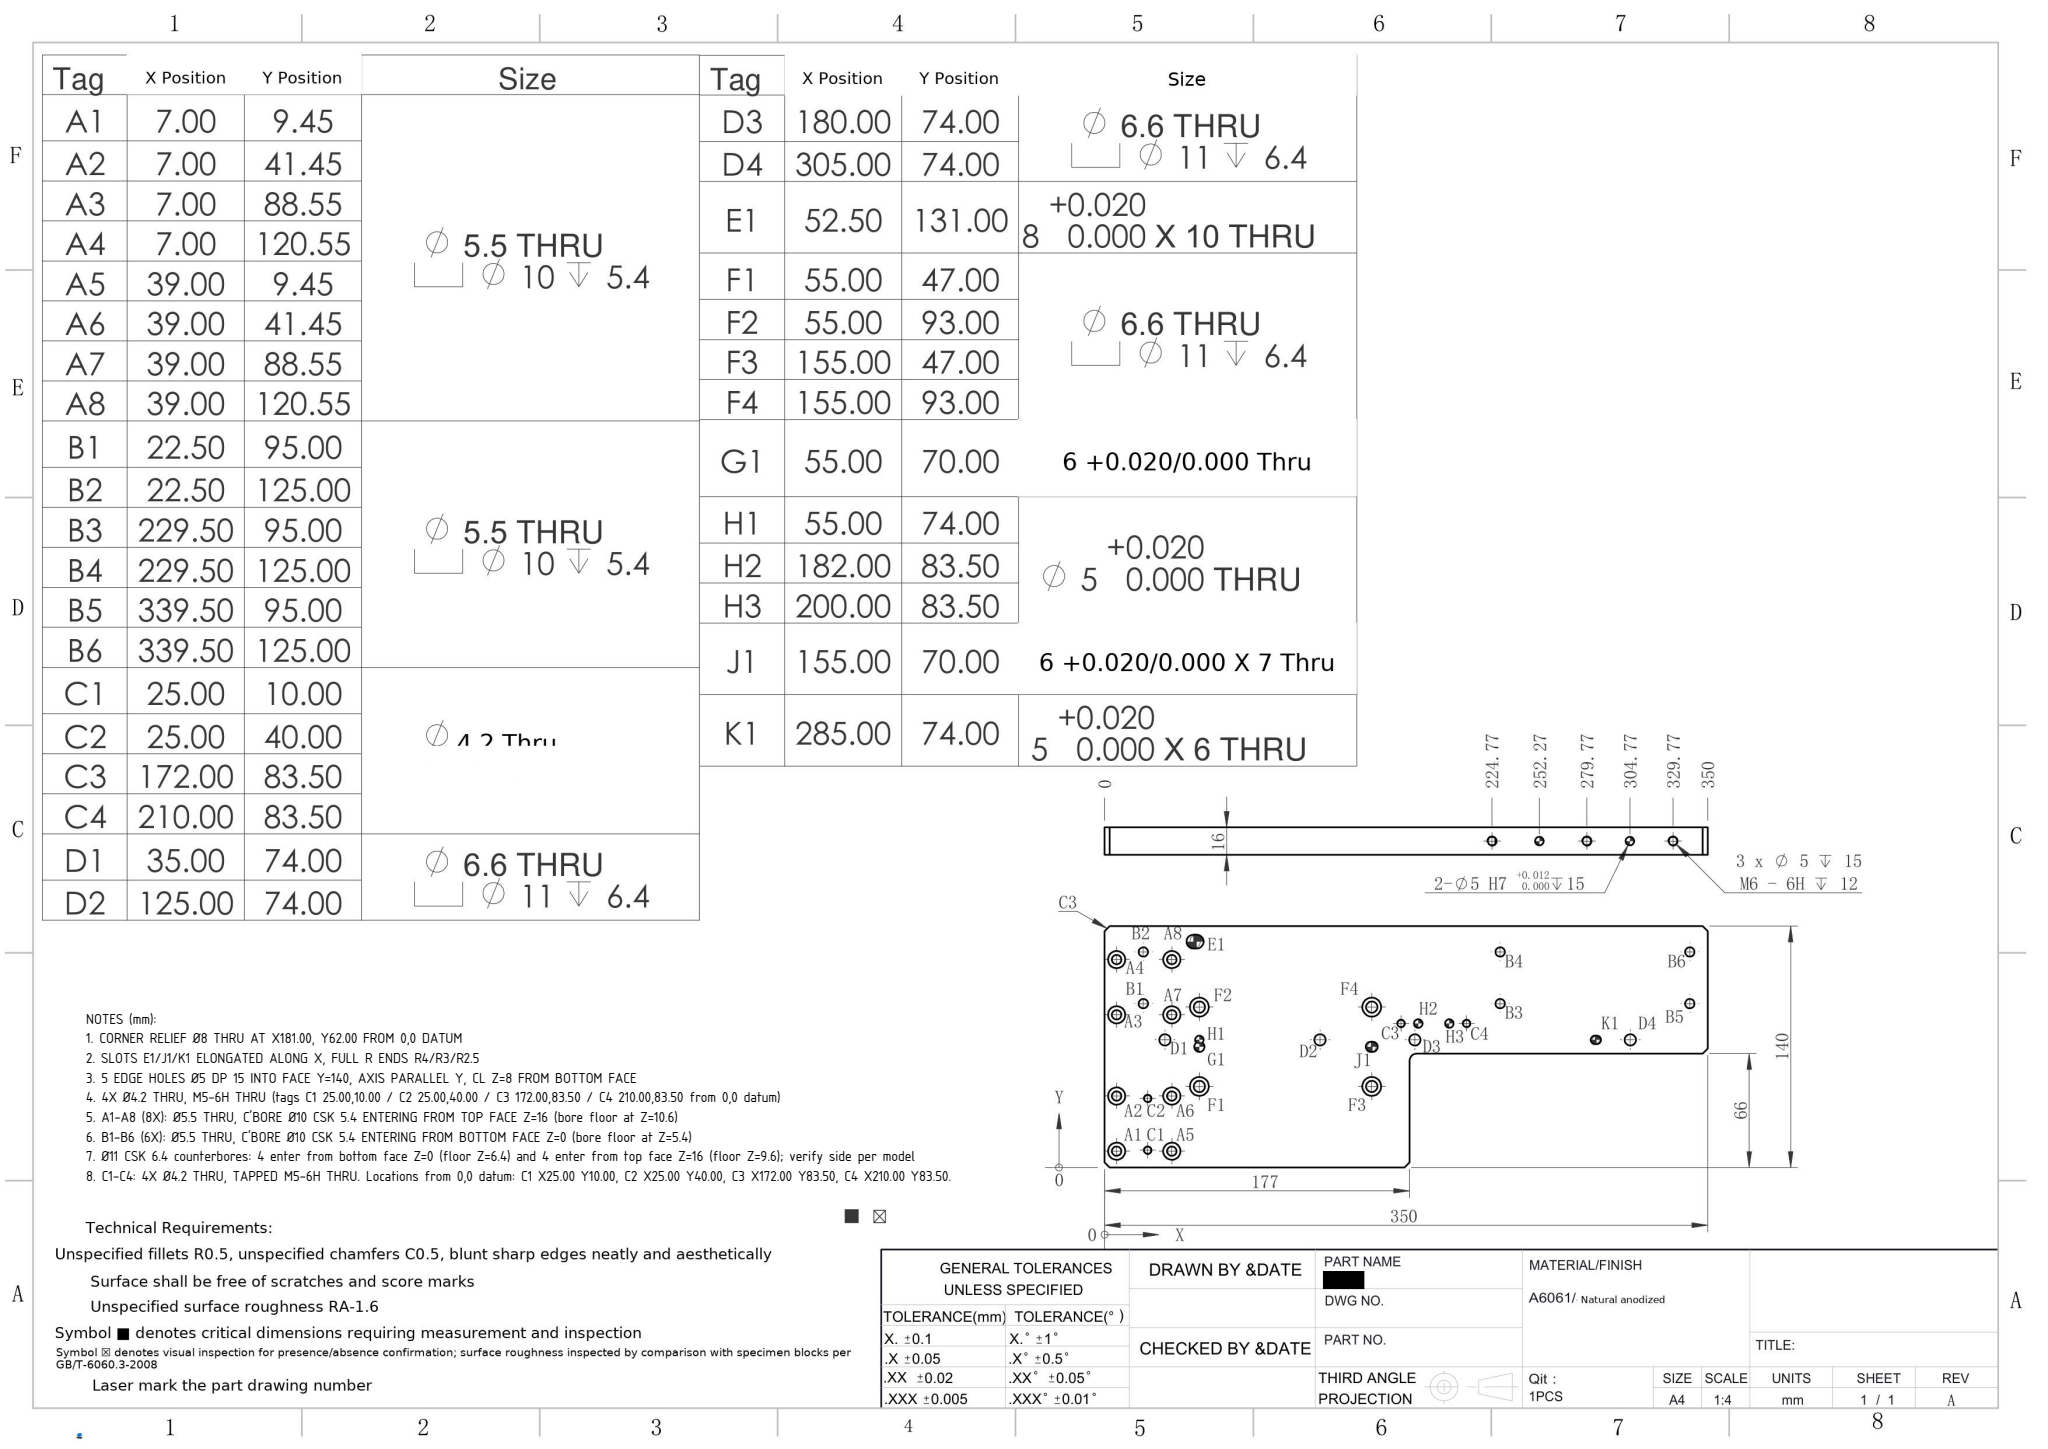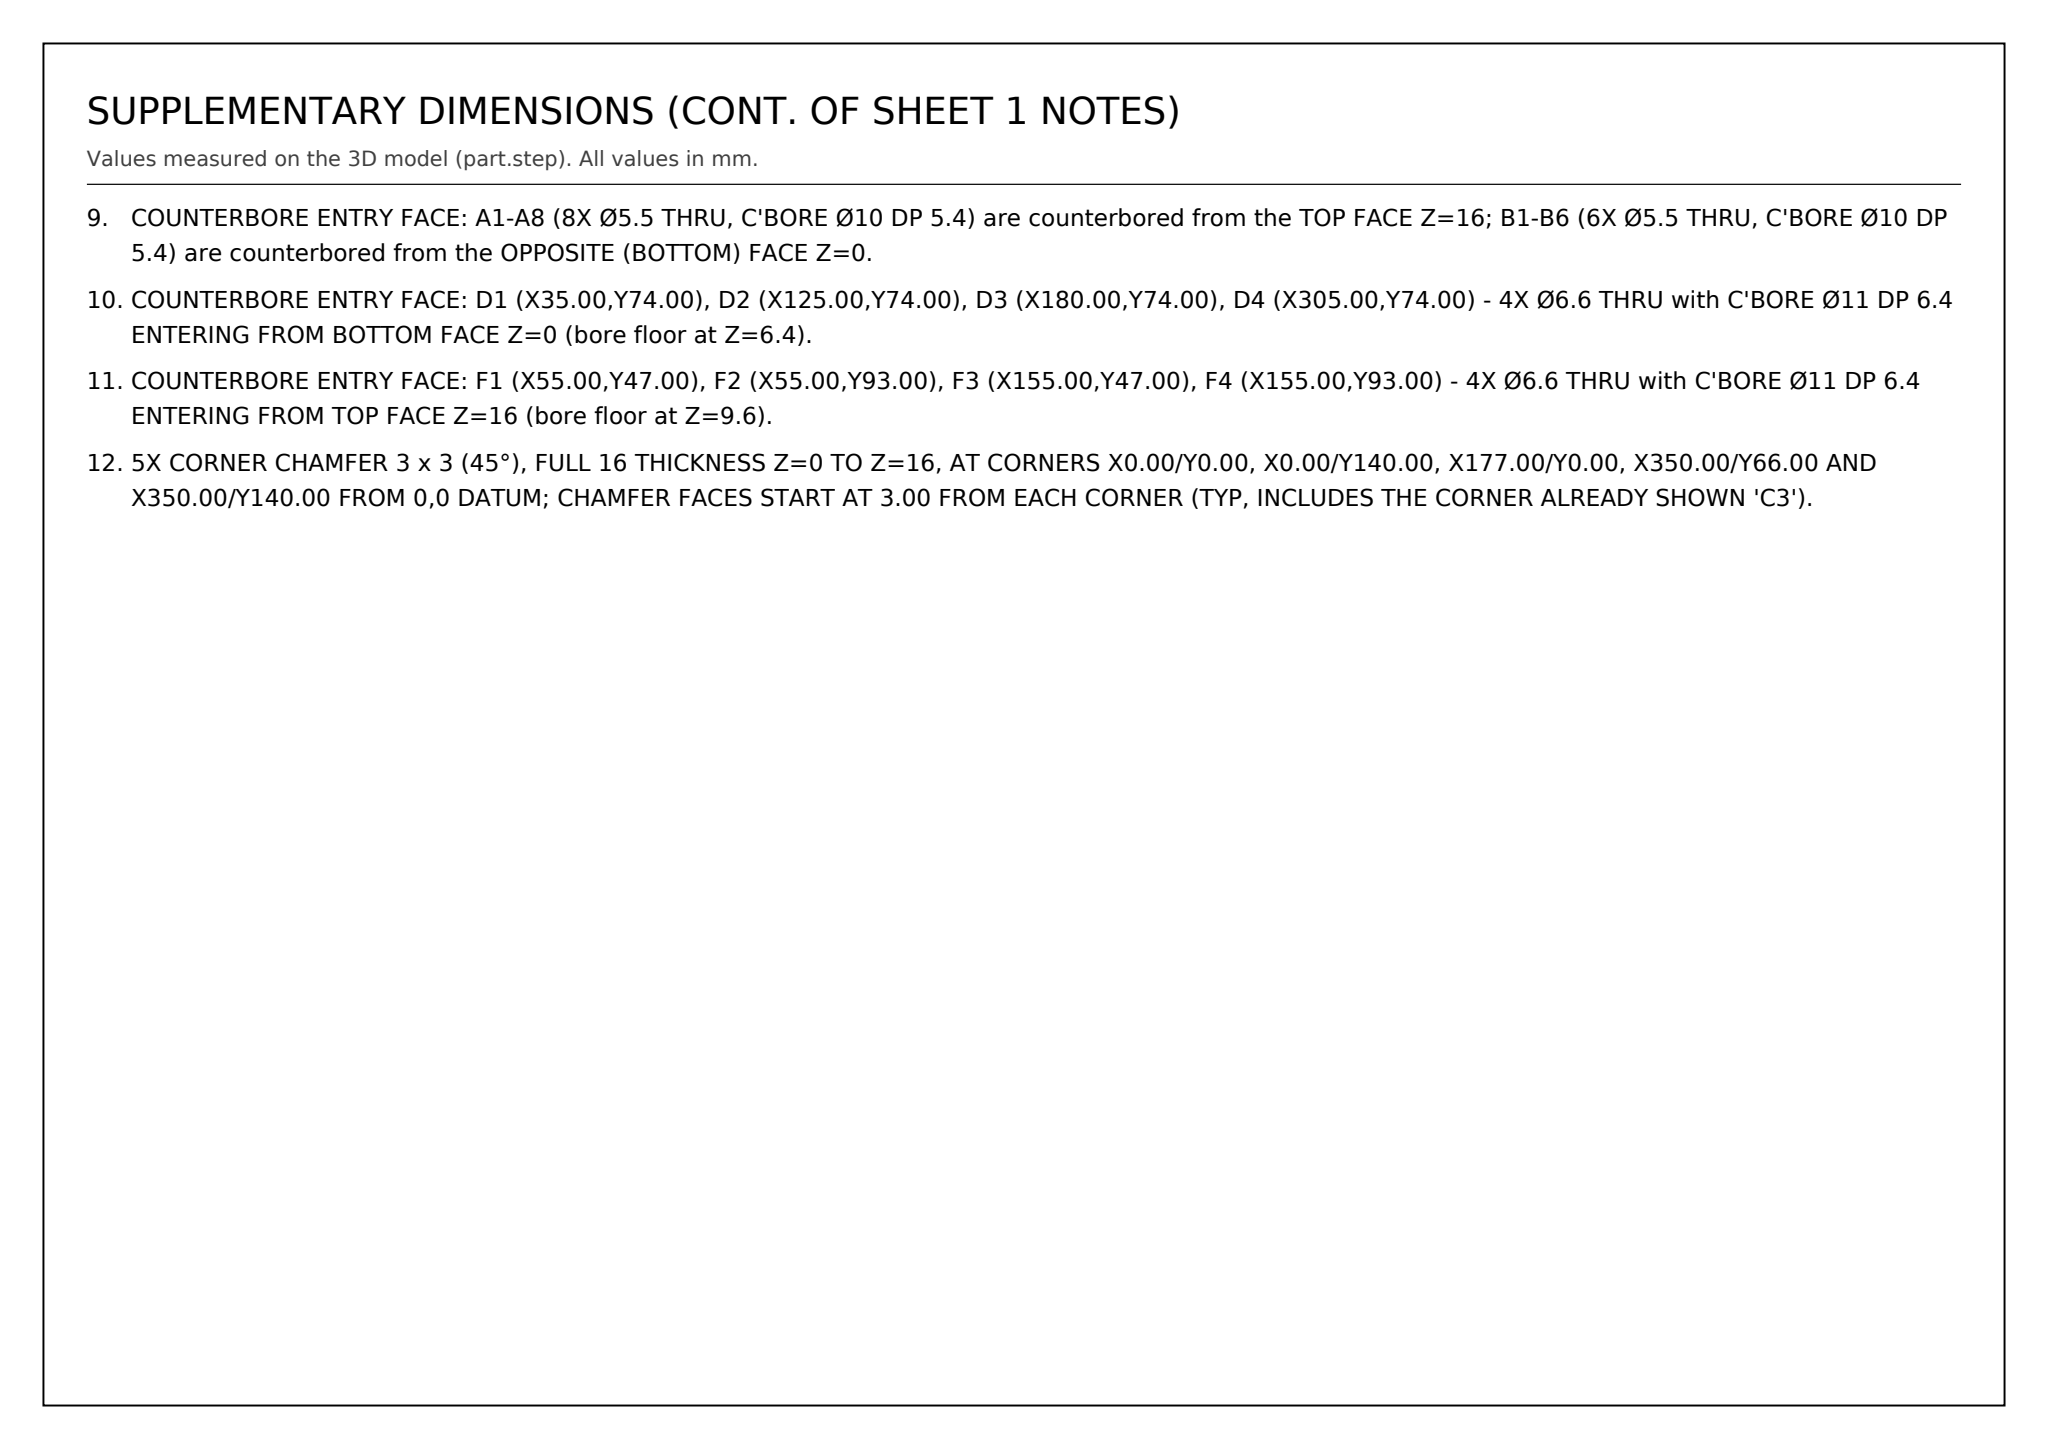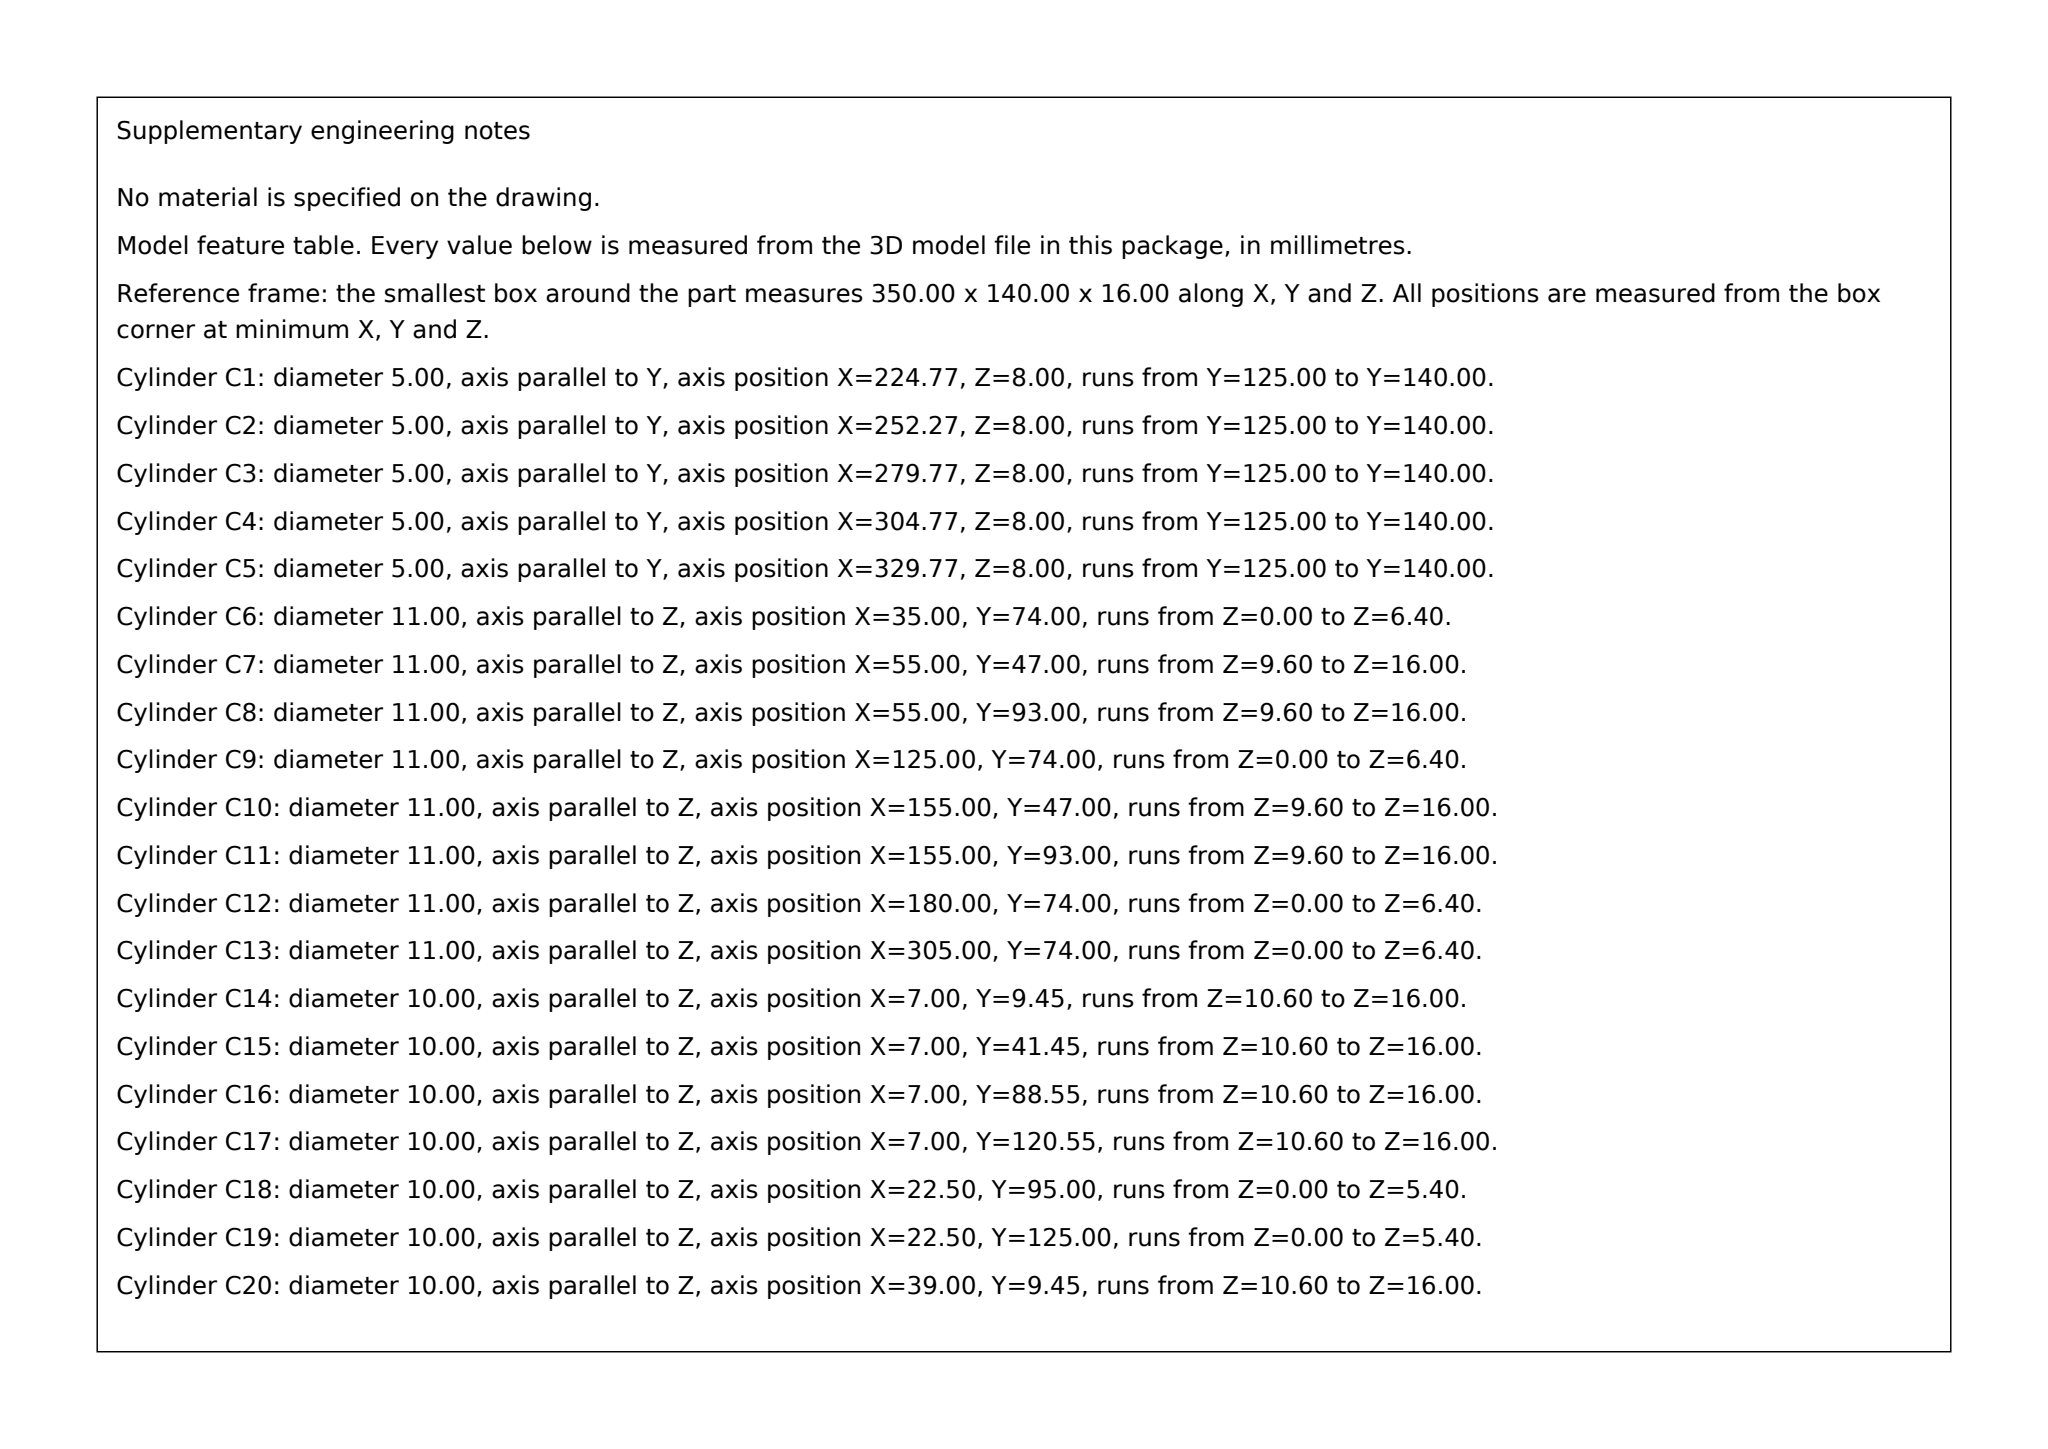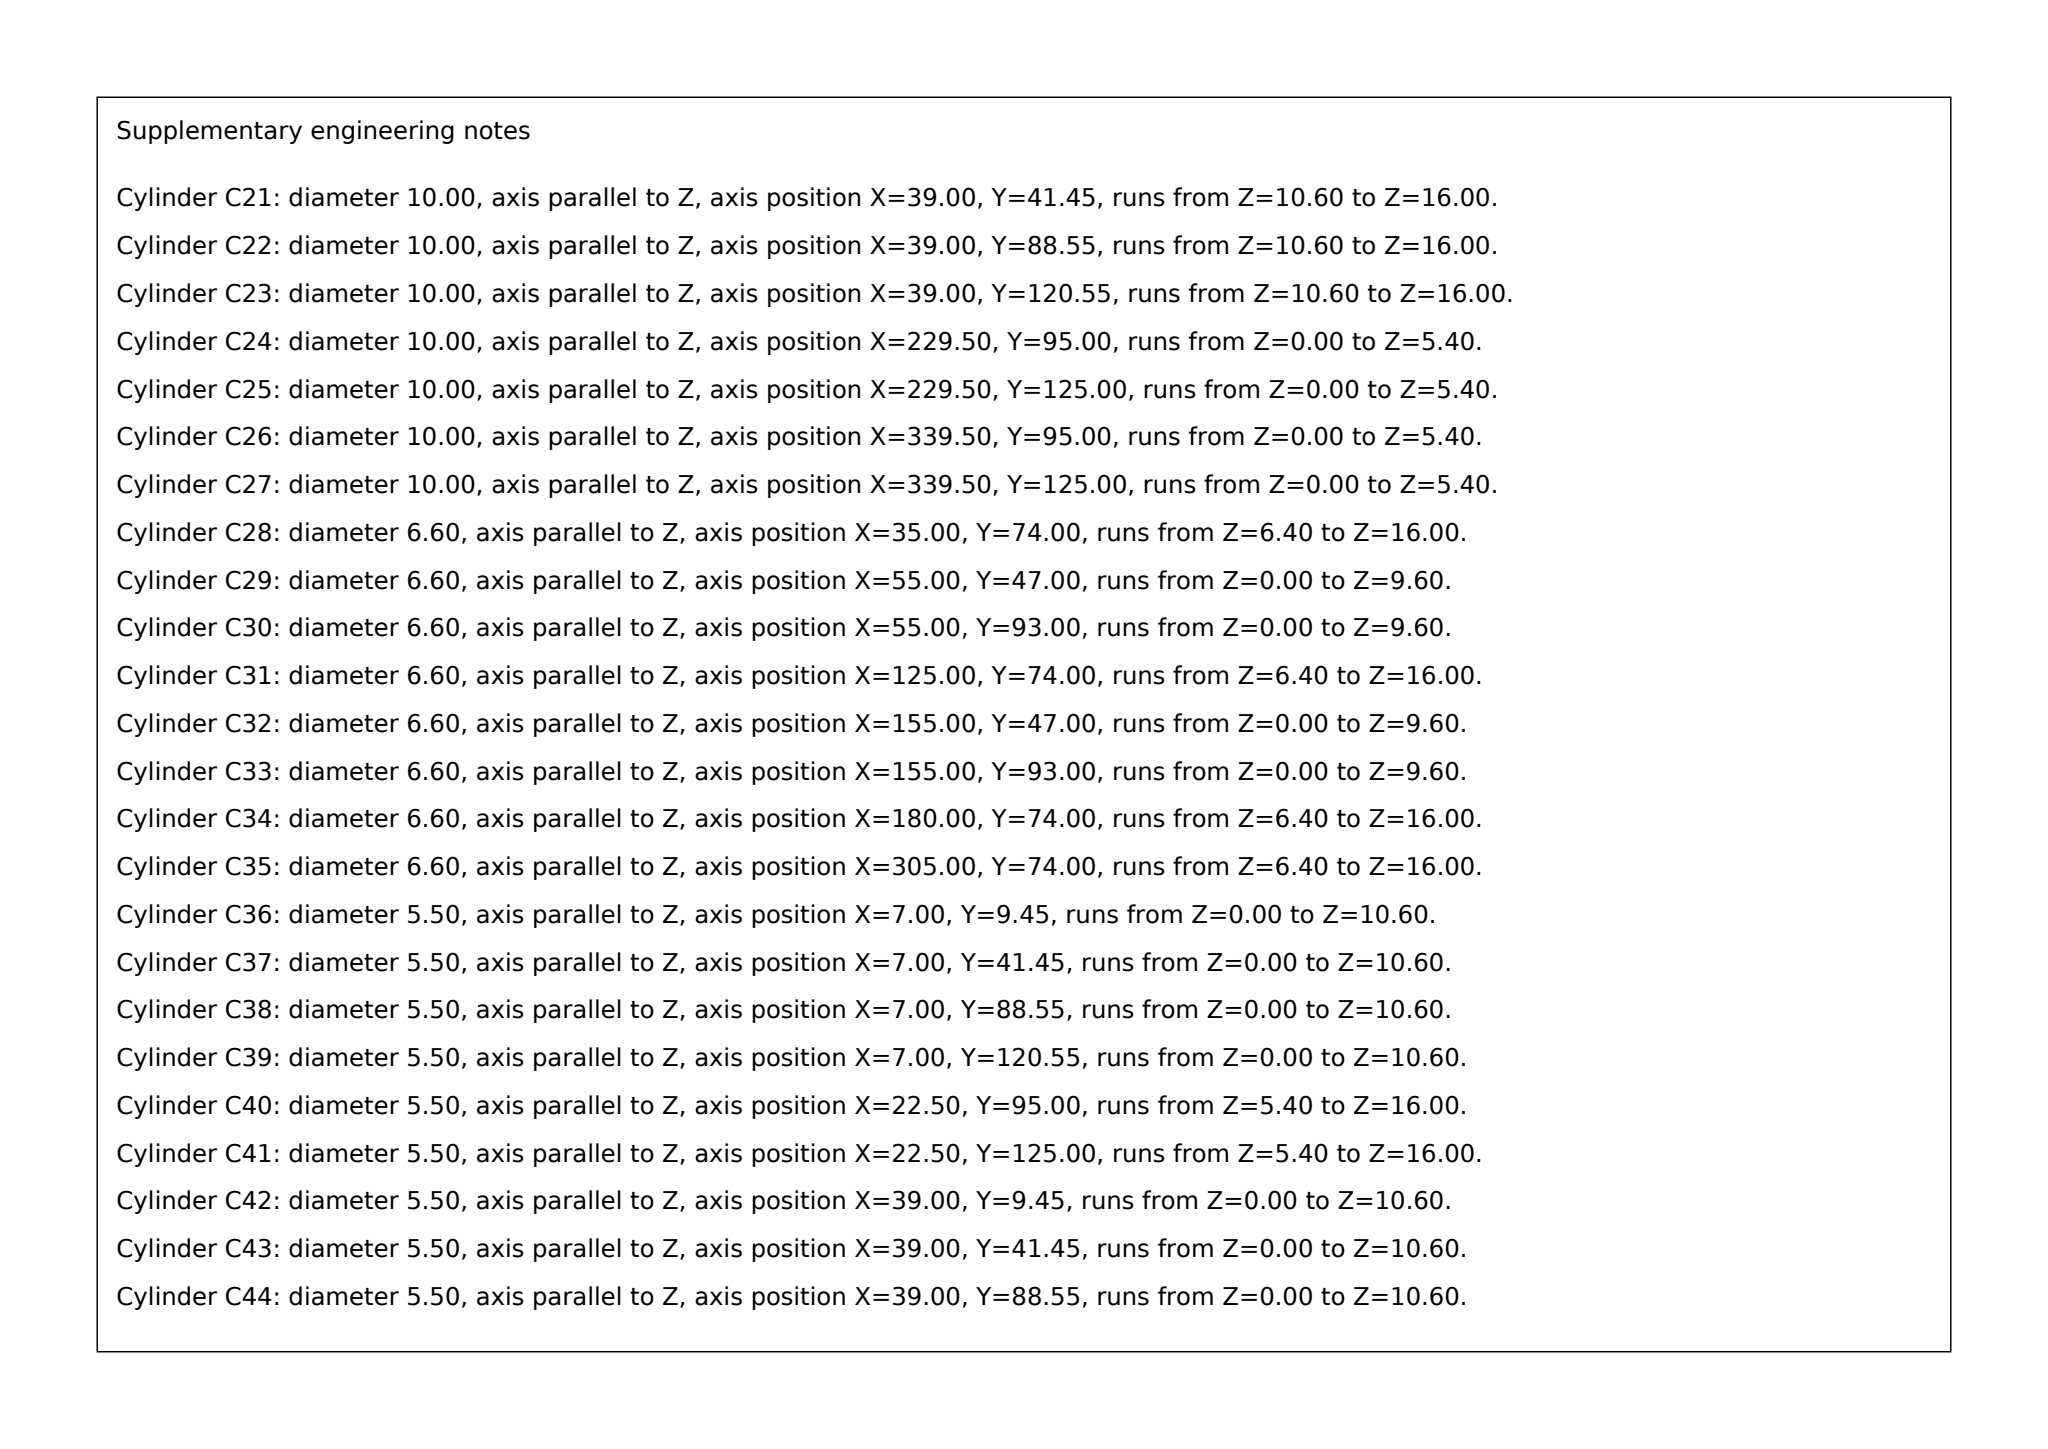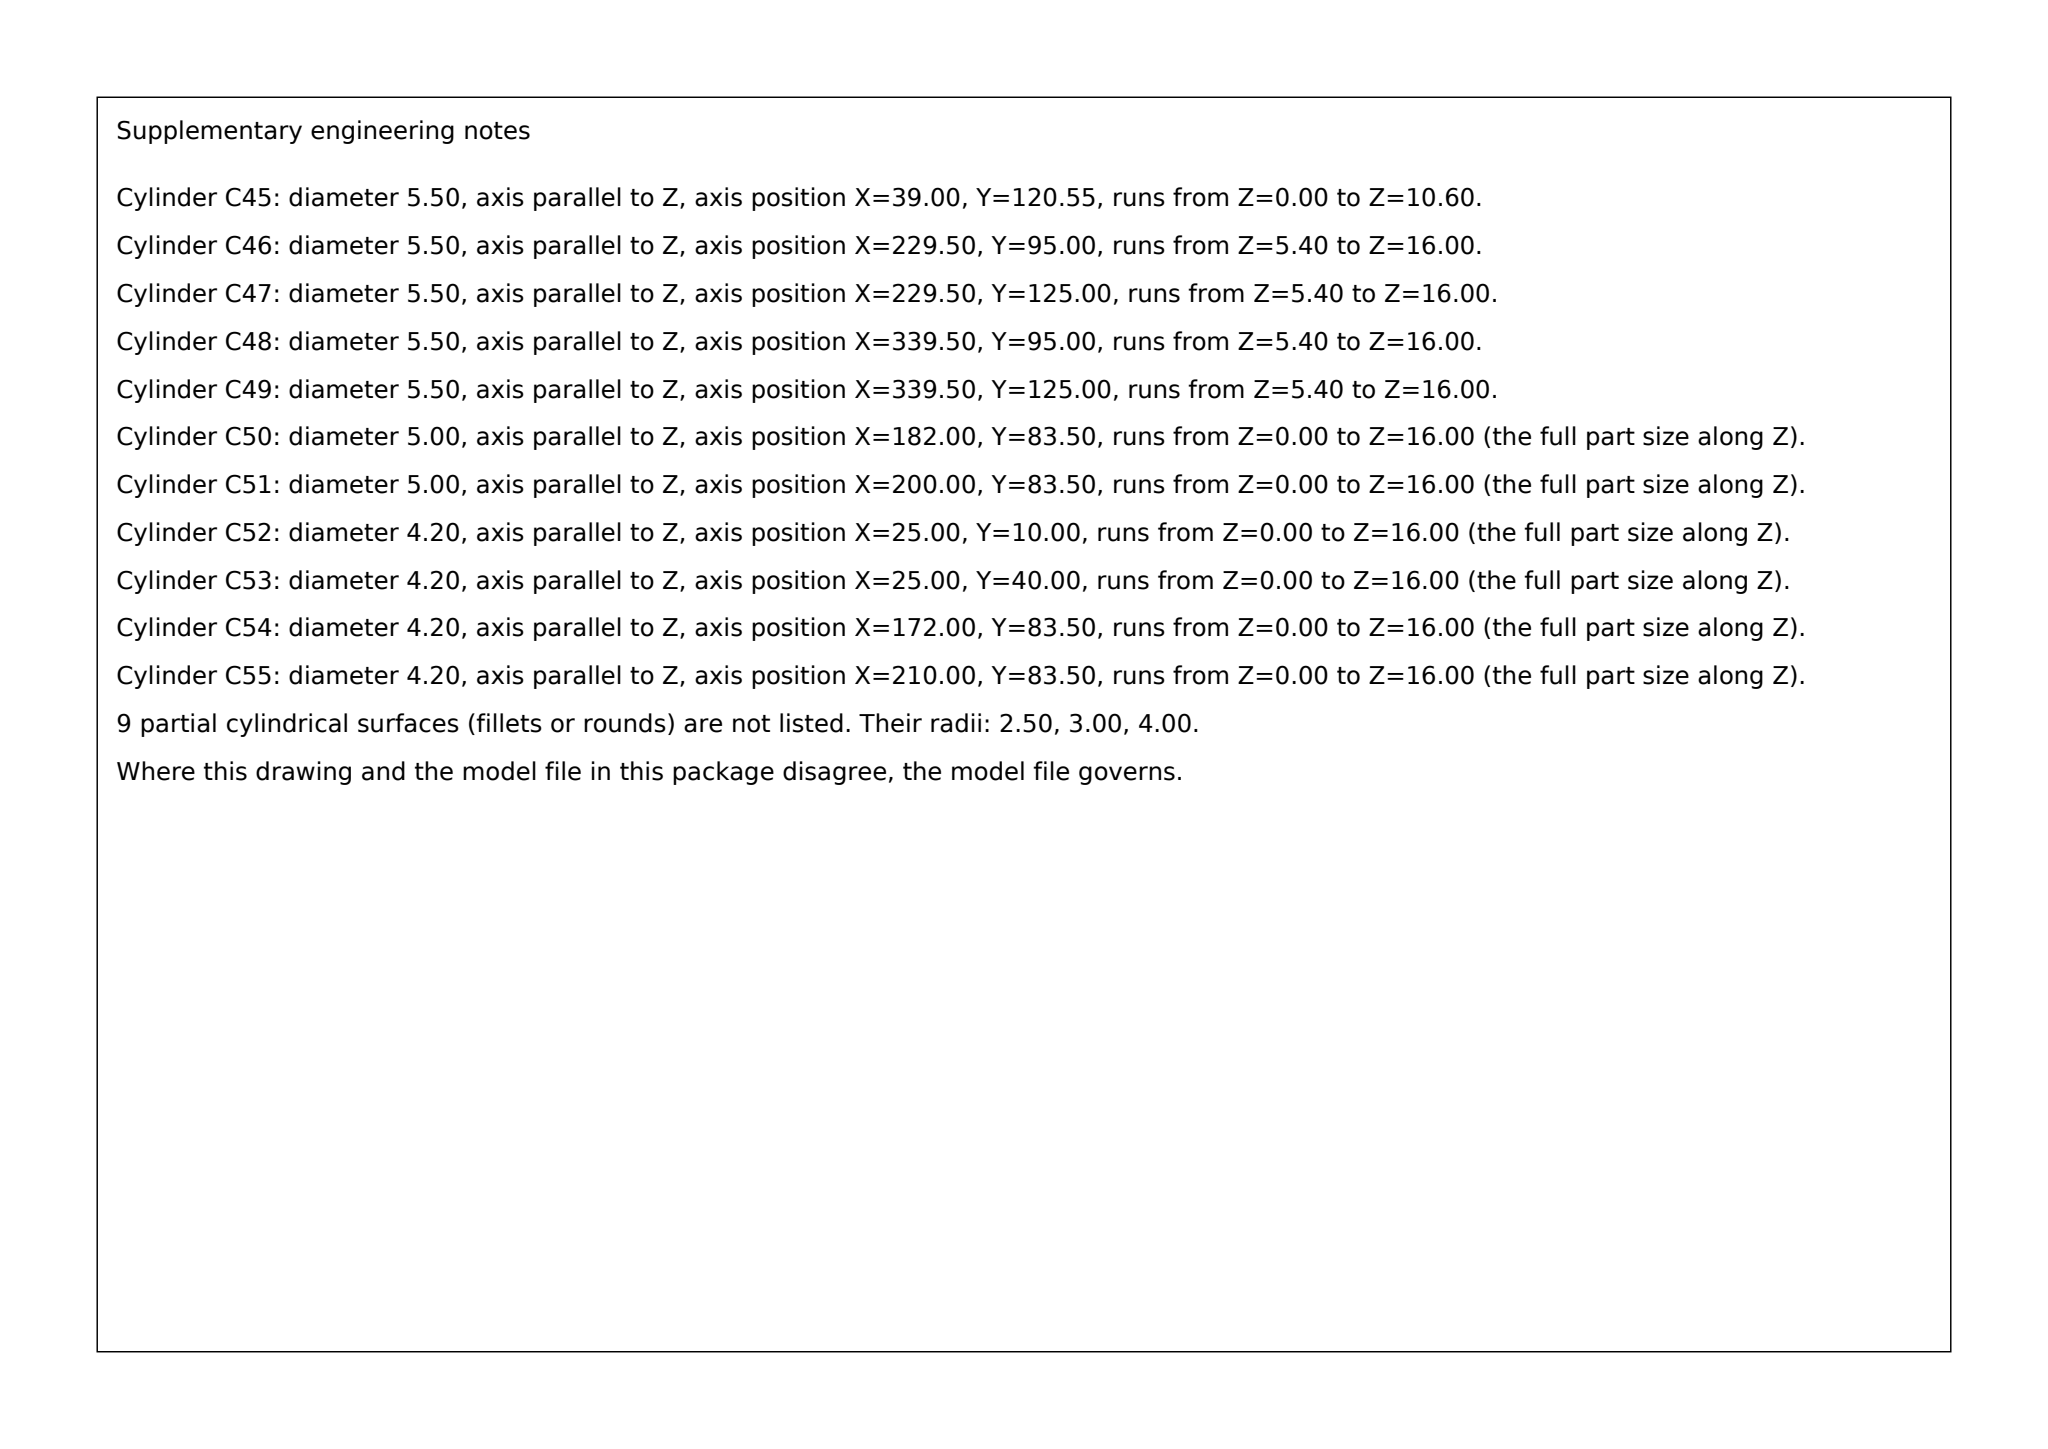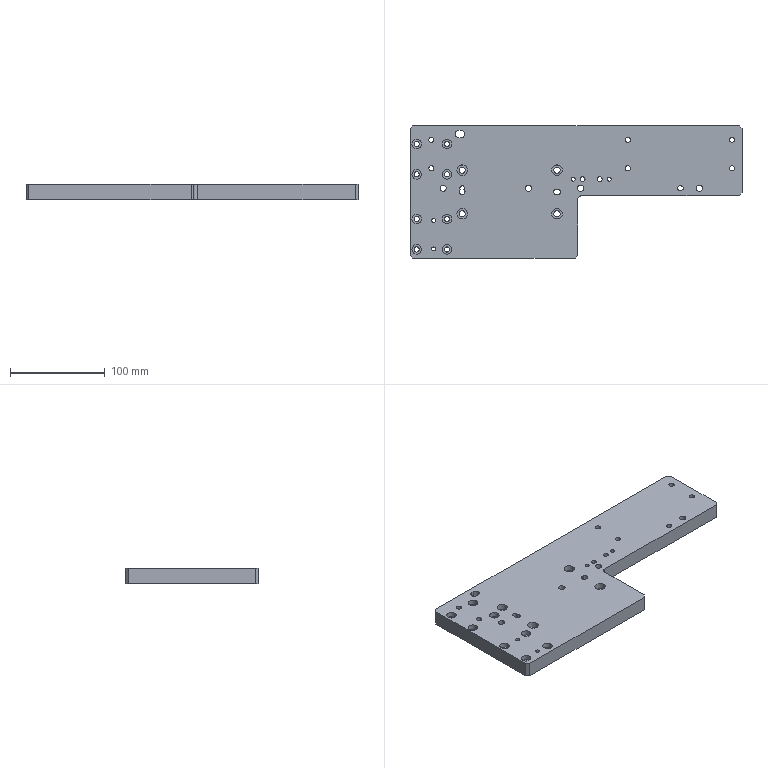Part | SolidWorks | mm | 1 solid | 177 faces | box 350 x 140 x 16 mm | volume 578307 mm3 | cylinder 126 | plane 41 | cone 10 | commonest cylinder face diameters 10 x28 5.5 x28 5 x20 11 x16 6.6 x16 4.2 x8 6 x6 8 x4
Drawing notes:
CORNER RELIEF Ø8 THRU AT X181.00, Y62.00 FROM 0,0 DATUM | from the solid: [8.0,'z',[181.0,62.0],16.0] = full 16 THK, at inside corner of 177/66 step
SLOTS E1/J1/K1 ELONGATED ALONG X, FULL R ENDS R4/R3/R2.5 | from the solid: Ø8 at x51.5&53.5 y131; Ø6 at x154.5&155.5 y70; Ø5 at x284.5&285.5 y74
5 EDGE HOLES Ø5 DP 15 INTO FACE Y=140, AXIS PARALLEL Y, CL Z=8 FROM BOTTOM FACE | from the solid: [5.0,'y',[224.77/252.27/279.77/304.77/329.77,null,8.0],15.0] in 16 THK plate
4X Ø4.2 THRU, M5-6H THRU (tags C1 25.00,10.00 / C2 25.00,40.00 / C3 172.00,83.50 / C4 210.00,83.50 from 0,0 datum) | from the solid: cylinders dia 4.2 axis z length 16.0 at (25,10),(25,40),(172,83.5),(210,83.5) with 118° cone ref dia 5.0
A1-A8 (8X): Ø5.5 THRU, C'BORE Ø10 CSK 5.4 ENTERING FROM TOP FACE Z=16 (bore floor at Z=10.6) | from the solid: axis_plane z=10.6 count 8 = floors of the eight Ø10x5.4 counterbores at the A1-A8 coordinates
B1-B6 (6X): Ø5.5 THRU, C'BORE Ø10 CSK 5.4 ENTERING FROM BOTTOM FACE Z=0 (bore floor at Z=5.4) | from the solid: axis_plane z=5.4 count 6 = floors of the six Ø10x5.4 counterbores at the B1-B6 coordinates
Ø11 CSK 6.4 counterbores: 4 enter from bottom face Z=0 (floor Z=6.4) and 4 enter from top face Z=16 (floor Z=9.6); verify side per model | from the solid: axis_planes z=6.4 count 4 and z=9.6 count 4 with eight Ø11x6.4 cylinders (D1-D4, F1-F4)
C1-C4: 4X Ø4.2 THRU, TAPPED M5-6H THRU. Locations from 0,0 datum: C1 X25.00 Y10.00, C2 X25.00 Y40.00, C3 X172.00 Y83.50, C4 X210.00 Y83.50. | from the solid: cylinders dia 4.2, axis z, length 16.0 (full 16 mm thickness) at (25,10), (25,40), (172,83.5), (210,83.5)
COUNTERBORE ENTRY FACE: A1-A8 (8X Ø5.5 THRU, C'BORE Ø10 DP 5.4) are counterbored from the TOP FACE Z=16; B1-B6 (6X Ø5.5 THRU, C'BORE Ø10 DP 5.4) are counterbored from the OPPOSITE (BOTTOM) FACE Z=0. | from the solid: dia 10 x 5.4 counterbores: axis-planes z=10.6 count 8 (bores entering from z=16, matches 8 A-holes) and z=5.4 count 6 (bores entering from z=0, matches 6 B-holes); Ø5.5 pilots length 10.6
COUNTERBORE ENTRY FACE: D1 (X35.00,Y74.00), D2 (X125.00,Y74.00), D3 (X180.00,Y74.00), D4 (X305.00,Y74.00) - 4X Ø6.6 THRU with C'BORE Ø11 DP 6.4 ENTERING FROM BOTTOM FACE Z=0 (bore floor at Z=6.4). | from the solid: cylinders: hole/bore Ø11 z-axis at (35,74),(125,74),(180,74),(305,74) from 0.0 to 6.4; Ø6.6 same XY from 6.4 to 16.0; planes z=6.4 at those XY
COUNTERBORE ENTRY FACE: F1 (X55.00,Y47.00), F2 (X55.00,Y93.00), F3 (X155.00,Y47.00), F4 (X155.00,Y93.00) - 4X Ø6.6 THRU with C'BORE Ø11 DP 6.4 ENTERING FROM TOP FACE Z=16 (bore floor at Z=9.6). | from the solid: cylinders: hole/bore Ø11 z-axis at (55,47),(55,93),(155,47),(155,93) from 9.6 to 16.0; Ø6.6 same XY from 0.0 to 9.6; planes z=9.6 at those XY
5X CORNER CHAMFER 3 x 3 (45°), FULL 16 THICKNESS Z=0 TO Z=16, AT CORNERS X0.00/Y0.00, X0.00/Y140.00, X177.00/Y0.00, X350.00/Y66.00 AND X350.00/Y140.00 FROM 0,0 DATUM; CHAMFER FACES START AT 3.00 FROM EACH CORNER (TYP, INCLUDES THE CORNER ALREADY SHOWN 'C3'). | from the solid: inclined_planes(chamfers/angled faces): five 45°/45°/90° faces, size 3.0 x 3.0 x 16.0, bbox_from [0,0,0], [0,137,0], [174,0,0], [347,137,0], [347,66,0]; bbox_xyz 350 x 140 x 16